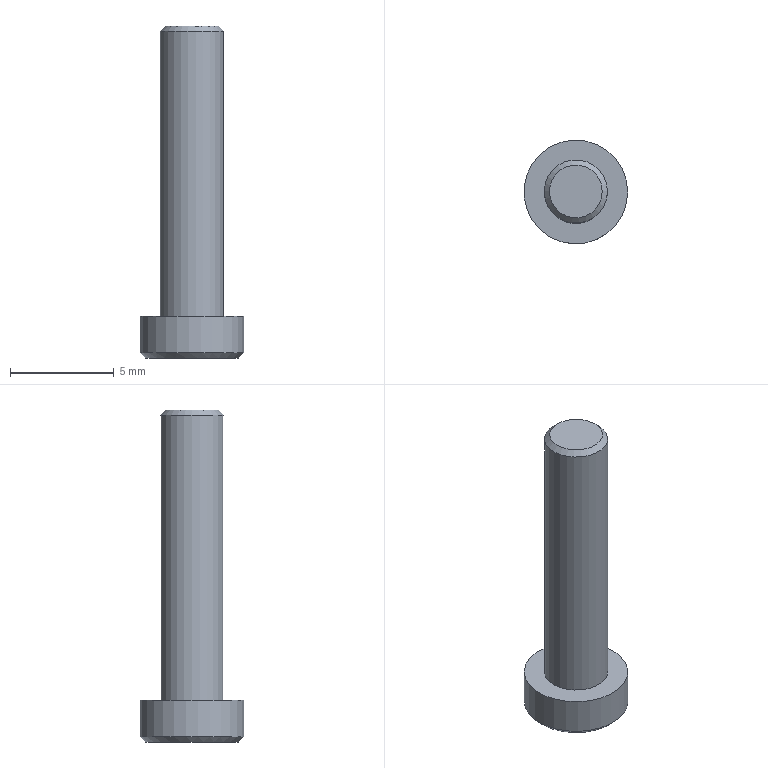Component | NX | SCREW_M3X12PRT_2 | 1 solid | 14 faces | volume 125 mm3 | plane 10 | cylinder 2 | cone 2 | commonest cylinder face diameters 3.045 x1 5 x1